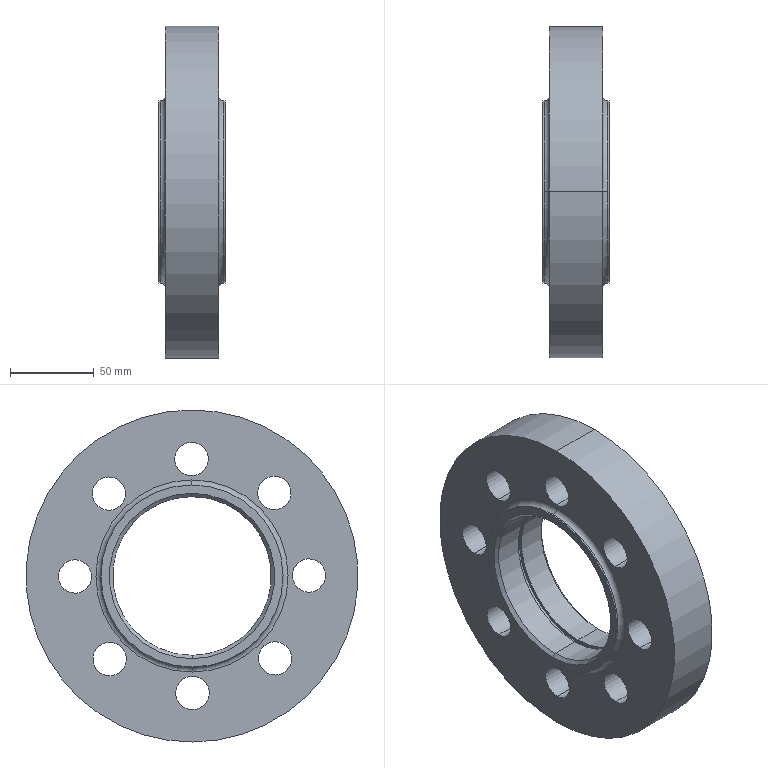Component | SolidWorks | SynchronousDrivenPulley-1 | 1 solid | 42 faces | volume 701473 mm3 | cylinder 28 | plane 6 | cone 4 | torus 4 | commonest cylinder face diameters 20 x16 95 x4 109 x4 98.5 x2 198.68 x2